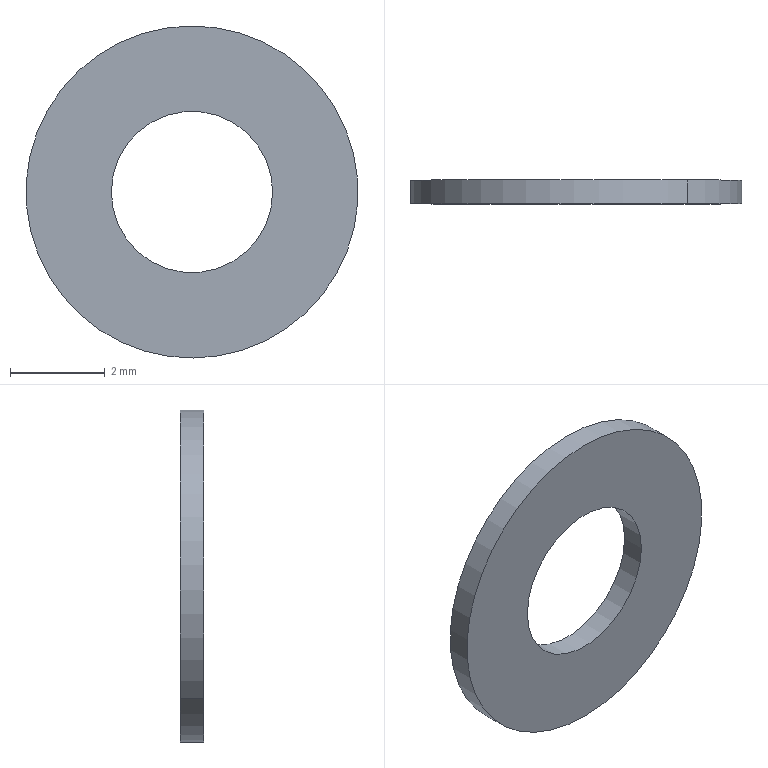Component | SolidWorks | GB_T95-2002FlatWasherC-grade3x0.5-33 | 1 solid | 6 faces | box 7 x 0.5 x 7 mm | volume 15 mm3 | cylinder 4 | plane 2 | commonest cylinder face diameters 7 x2 3.4 x2
build123d program:
from build123d import *

# Parameters (mm, degrees)
SKETCH1_W = 1.8
SKETCH1_H = 0.5


with BuildPart() as part:
    # Sketch1 → Base-Revolve (revolve)
    with BuildSketch(Plane.XY, mode=Mode.PRIVATE) as base_revolve_sk:
        with Locations((-2.6, 8.895)):
            Rectangle(SKETCH1_W, SKETCH1_H)
    revolve(base_revolve_sk.sketch.rotate(Axis((0, 0, 0), (0, 1, 0)), 270), axis=Axis((0, 0, 0), (0, 1, 0)))


solid = part.part

# Placed as in the assembly
solid = solid.moved(Location((-16.097, -0.8355, 28), (0, 0, 0)))
STEP:
#1=CARTESIAN_POINT('',(-0.7265,0.3271,1.));
#2=VERTEX_POINT('',#1);
#3=CARTESIAN_POINT('',(-0.541,0.3271,1.204));
#4=VERTEX_POINT('',#3);
#5=CARTESIAN_POINT('',(-0.6337,0.3271,1.102));
#6=DIRECTION('',(0.,-1.,-0.));
#7=DIRECTION('',(-0.6731,0.,-0.7395));
#8=AXIS2_PLACEMENT_3D('',#5,#6,#7);
#9=CIRCLE('',#8,0.1378);
#10=EDGE_CURVE('',#2,#4,#9,.T.);
#11=ORIENTED_EDGE('',*,*,#10,.T.);
#12=CARTESIAN_POINT('',(-0.541,0.3074,1.204));
#13=VERTEX_POINT('',#12);
#14=CARTESIAN_POINT('',(-0.541,-0.0329,1.204));
#15=DIRECTION('',(0.,-1.,-0.));
#16=VECTOR('',#15,39.37);
#17=LINE('',#14,#16);
#18=EDGE_CURVE('',#4,#13,#17,.T.);
#19=ORIENTED_EDGE('',*,*,#18,.T.);
#20=CARTESIAN_POINT('',(-0.7265,0.3074,1.));
#21=VERTEX_POINT('',#20);
#22=CARTESIAN_POINT('',(-0.6337,0.3074,1.102));
#23=DIRECTION('',(0.,-1.,-0.));
#24=DIRECTION('',(-0.6731,0.,-0.7395));
#25=AXIS2_PLACEMENT_3D('',#22,#23,#24);
#26=CIRCLE('',#25,0.1378);
#27=EDGE_CURVE('',#21,#13,#26,.T.);
#28=ORIENTED_EDGE('',*,*,#27,.F.);
#29=CARTESIAN_POINT('',(-0.7265,-0.0329,1.));
#30=DIRECTION('',(0.,-1.,-0.));
#31=VECTOR('',#30,39.37);
#32=LINE('',#29,#31);
#33=EDGE_CURVE('',#2,#21,#32,.T.);
#34=ORIENTED_EDGE('',*,*,#33,.F.);
#35=EDGE_LOOP('',(#11,#19,#28,#34));
#36=FACE_OUTER_BOUND('',#35,.T.);
#37=CARTESIAN_POINT('',(-0.6337,-0.0329,1.102));
#38=DIRECTION('',(0.,-1.,-0.));
#39=DIRECTION('',(-0.6731,0.,-0.7395));
#40=AXIS2_PLACEMENT_3D('',#37,#38,#39);
#41=CYLINDRICAL_SURFACE('',#40,0.1378);
#42=ADVANCED_FACE('',(#36),#41,.T.);
#43=CARTESIAN_POINT('',(-0.5887,0.3271,1.152));
#44=VERTEX_POINT('',#43);
#45=CARTESIAN_POINT('',(-0.6788,0.3271,1.053));
#46=VERTEX_POINT('',#45);
#47=CARTESIAN_POINT('',(-0.6337,0.3271,1.102));
#48=DIRECTION('',(0.,-1.,-0.));
#49=DIRECTION('',(-0.6731,0.,-0.7395));
#50=AXIS2_PLACEMENT_3D('',#47,#48,#49);
#51=CIRCLE('',#50,0.06693);
#52=EDGE_CURVE('',#44,#46,#51,.T.);
#53=ORIENTED_EDGE('',*,*,#52,.F.);
#54=CARTESIAN_POINT('',(-0.5887,0.3074,1.152));
#55=VERTEX_POINT('',#54);
#56=CARTESIAN_POINT('',(-0.5887,-0.0329,1.152));
#57=DIRECTION('',(0.,-1.,-0.));
#58=VECTOR('',#57,39.37);
#59=LINE('',#56,#58);
#60=EDGE_CURVE('',#44,#55,#59,.T.);
#61=ORIENTED_EDGE('',*,*,#60,.T.);
#62=CARTESIAN_POINT('',(-0.6788,0.3074,1.053));
#63=VERTEX_POINT('',#62);
#64=CARTESIAN_POINT('',(-0.6337,0.3074,1.102));
#65=DIRECTION('',(0.,-1.,-0.));
#66=DIRECTION('',(-0.6731,0.,-0.7395));
#67=AXIS2_PLACEMENT_3D('',#64,#65,#66);
#68=CIRCLE('',#67,0.06693);
#69=EDGE_CURVE('',#55,#63,#68,.T.);
#70=ORIENTED_EDGE('',*,*,#69,.T.);
#71=CARTESIAN_POINT('',(-0.6788,-0.0329,1.053));
#72=DIRECTION('',(0.,-1.,-0.));
#73=VECTOR('',#72,39.37);
#74=LINE('',#71,#73);
#75=EDGE_CURVE('',#46,#63,#74,.T.);
#76=ORIENTED_EDGE('',*,*,#75,.F.);
#77=EDGE_LOOP('',(#53,#61,#70,#76));
#78=FACE_OUTER_BOUND('',#77,.T.);
#79=CARTESIAN_POINT('',(-0.6337,-0.0329,1.102));
#80=DIRECTION('',(0.,-1.,-0.));
#81=DIRECTION('',(-0.6731,0.,-0.7395));
#82=AXIS2_PLACEMENT_3D('',#79,#80,#81);
#83=CYLINDRICAL_SURFACE('',#82,0.06693);
#84=ADVANCED_FACE('',(#78),#83,.F.);
#85=ORIENTED_EDGE('',*,*,#60,.F.);
#86=CARTESIAN_POINT('',(-0.6337,0.3271,1.102));
#87=DIRECTION('',(0.,-1.,-0.));
#88=DIRECTION('',(-0.6731,0.,-0.7395));
#89=AXIS2_PLACEMENT_3D('',#86,#87,#88);
#90=CIRCLE('',#89,0.06693);
#91=EDGE_CURVE('',#46,#44,#90,.T.);
#92=ORIENTED_EDGE('',*,*,#91,.F.);
#93=ORIENTED_EDGE('',*,*,#75,.T.);
#94=CARTESIAN_POINT('',(-0.6337,0.3074,1.102));
#95=DIRECTION('',(0.,-1.,-0.));
#96=DIRECTION('',(-0.6731,0.,-0.7395));
#97=AXIS2_PLACEMENT_3D('',#94,#95,#96);
#98=CIRCLE('',#97,0.06693);
#99=EDGE_CURVE('',#63,#55,#98,.T.);
#100=ORIENTED_EDGE('',*,*,#99,.T.);
#101=EDGE_LOOP('',(#85,#92,#93,#100));
#102=FACE_OUTER_BOUND('',#101,.T.);
#103=CARTESIAN_POINT('',(-0.6337,-0.0329,1.102));
#104=DIRECTION('',(0.,-1.,-0.));
#105=DIRECTION('',(-0.6731,0.,-0.7395));
#106=AXIS2_PLACEMENT_3D('',#103,#104,#105);
#107=CYLINDRICAL_SURFACE('',#106,0.06693);
#108=ADVANCED_FACE('',(#102),#107,.F.);
#109=ORIENTED_EDGE('',*,*,#10,.F.);
#110=CARTESIAN_POINT('',(-0.6337,0.3271,1.102));
#111=DIRECTION('',(0.,-1.,-0.));
#112=DIRECTION('',(-0.6731,0.,-0.7395));
#113=AXIS2_PLACEMENT_3D('',#110,#111,#112);
#114=CIRCLE('',#113,0.1378);
#115=EDGE_CURVE('',#4,#2,#114,.T.);
#116=ORIENTED_EDGE('',*,*,#115,.F.);
#117=EDGE_LOOP('',(#109,#116));
#118=FACE_OUTER_BOUND('',#117,.T.);
#119=ORIENTED_EDGE('',*,*,#91,.T.);
#120=ORIENTED_EDGE('',*,*,#52,.T.);
#121=EDGE_LOOP('',(#119,#120));
#122=FACE_BOUND('',#121,.T.);
#123=CARTESIAN_POINT('',(-0.6832,0.3271,1.147));
#124=DIRECTION('',(0.,-1.,-0.));
#125=DIRECTION('',(-0.6731,0.,-0.7395));
#126=AXIS2_PLACEMENT_3D('',#123,#124,#125);
#127=PLANE('',#126);
#128=ADVANCED_FACE('',(#118,#122),#127,.F.);
#129=ORIENTED_EDGE('',*,*,#18,.F.);
#130=ORIENTED_EDGE('',*,*,#115,.T.);
#131=ORIENTED_EDGE('',*,*,#33,.T.);
#132=CARTESIAN_POINT('',(-0.6337,0.3074,1.102));
#133=DIRECTION('',(0.,-1.,-0.));
#134=DIRECTION('',(-0.6731,0.,-0.7395));
#135=AXIS2_PLACEMENT_3D('',#132,#133,#134);
#136=CIRCLE('',#135,0.1378);
#137=EDGE_CURVE('',#13,#21,#136,.T.);
#138=ORIENTED_EDGE('',*,*,#137,.F.);
#139=EDGE_LOOP('',(#129,#130,#131,#138));
#140=FACE_OUTER_BOUND('',#139,.T.);
#141=CARTESIAN_POINT('',(-0.6337,-0.0329,1.102));
#142=DIRECTION('',(0.,-1.,-0.));
#143=DIRECTION('',(-0.6731,0.,-0.7395));
#144=AXIS2_PLACEMENT_3D('',#141,#142,#143);
#145=CYLINDRICAL_SURFACE('',#144,0.1378);
#146=ADVANCED_FACE('',(#140),#145,.T.);
#147=ORIENTED_EDGE('',*,*,#99,.F.);
#148=ORIENTED_EDGE('',*,*,#69,.F.);
#149=EDGE_LOOP('',(#147,#148));
#150=FACE_BOUND('',#149,.T.);
#151=ORIENTED_EDGE('',*,*,#27,.T.);
#152=ORIENTED_EDGE('',*,*,#137,.T.);
#153=EDGE_LOOP('',(#151,#152));
#154=FACE_OUTER_BOUND('',#153,.T.);
#155=CARTESIAN_POINT('',(-0.6832,0.3074,1.147));
#156=DIRECTION('',(-0.,1.,0.));
#157=DIRECTION('',(0.6731,-0.,0.7395));
#158=AXIS2_PLACEMENT_3D('',#155,#156,#157);
#159=PLANE('',#158);
#160=ADVANCED_FACE('',(#150,#154),#159,.F.);
#161=CLOSED_SHELL('',(#42,#84,#108,#128,#146,#160));
#162=MANIFOLD_SOLID_BREP('',#161);
#163=CARTESIAN_POINT('',(0.,0.,0.));
#164=DIRECTION('',(0.,0.,1.));
#165=DIRECTION('',(1.,0.,0.));
#166=AXIS2_PLACEMENT_3D('',#163,#164,#165);
#167=(LENGTH_UNIT()NAMED_UNIT(*)SI_UNIT($,.METRE.));
#168=LENGTH_MEASURE_WITH_UNIT(LENGTH_MEASURE(0.0254),#167);
#169=DIMENSIONAL_EXPONENTS(1.,0.,0.,0.,0.,0.,0.);
#170=(CONVERSION_BASED_UNIT('',#168)LENGTH_UNIT()NAMED_UNIT(#169));
#171=UNCERTAINTY_MEASURE_WITH_UNIT(LENGTH_MEASURE(0.00001),#170,'','');
#172=(NAMED_UNIT(*)PLANE_ANGLE_UNIT()SI_UNIT($,.RADIAN.));
#173=(NAMED_UNIT(*)SI_UNIT($,.STERADIAN.)SOLID_ANGLE_UNIT());
#174=(GEOMETRIC_REPRESENTATION_CONTEXT(3)GLOBAL_UNCERTAINTY_ASSIGNED_CONTEXT((#171))GLOBAL_UNIT_ASSIGNED_CONTEXT((#170,#172,#173))REPRESENTATION_CONTEXT('',''));
#175=ADVANCED_BREP_SHAPE_REPRESENTATION('',(#162,#166),#174);
#176=COLOUR_RGB('',0.7922,0.8196,0.9333);
#177=FILL_AREA_STYLE_COLOUR('',#176);
#178=FILL_AREA_STYLE('',(#177));
#179=SURFACE_STYLE_FILL_AREA(#178);
#180=SURFACE_SIDE_STYLE('',(#179));
#181=SURFACE_STYLE_USAGE(.BOTH.,#180);
#182=PRESENTATION_STYLE_ASSIGNMENT((#181));
#183=STYLED_ITEM('',(#182),#162);
#184=PRESENTATION_LAYER_ASSIGNMENT('','',(#183));
#185=(LENGTH_UNIT()NAMED_UNIT(*)SI_UNIT($,.METRE.));
#186=LENGTH_MEASURE_WITH_UNIT(LENGTH_MEASURE(0.0254),#185);
#187=DIMENSIONAL_EXPONENTS(1.,0.,0.,0.,0.,0.,0.);
#188=(CONVERSION_BASED_UNIT('',#186)LENGTH_UNIT()NAMED_UNIT(#187));
#189=UNCERTAINTY_MEASURE_WITH_UNIT(LENGTH_MEASURE(0.00001),#188,'','');
#190=(NAMED_UNIT(*)PLANE_ANGLE_UNIT()SI_UNIT($,.RADIAN.));
#191=(NAMED_UNIT(*)SI_UNIT($,.STERADIAN.)SOLID_ANGLE_UNIT());
#192=(GEOMETRIC_REPRESENTATION_CONTEXT(3)GLOBAL_UNCERTAINTY_ASSIGNED_CONTEXT((#189))GLOBAL_UNIT_ASSIGNED_CONTEXT((#188,#190,#191))REPRESENTATION_CONTEXT('',''));
#193=MECHANICAL_DESIGN_GEOMETRIC_PRESENTATION_REPRESENTATION('',(#183),#192);